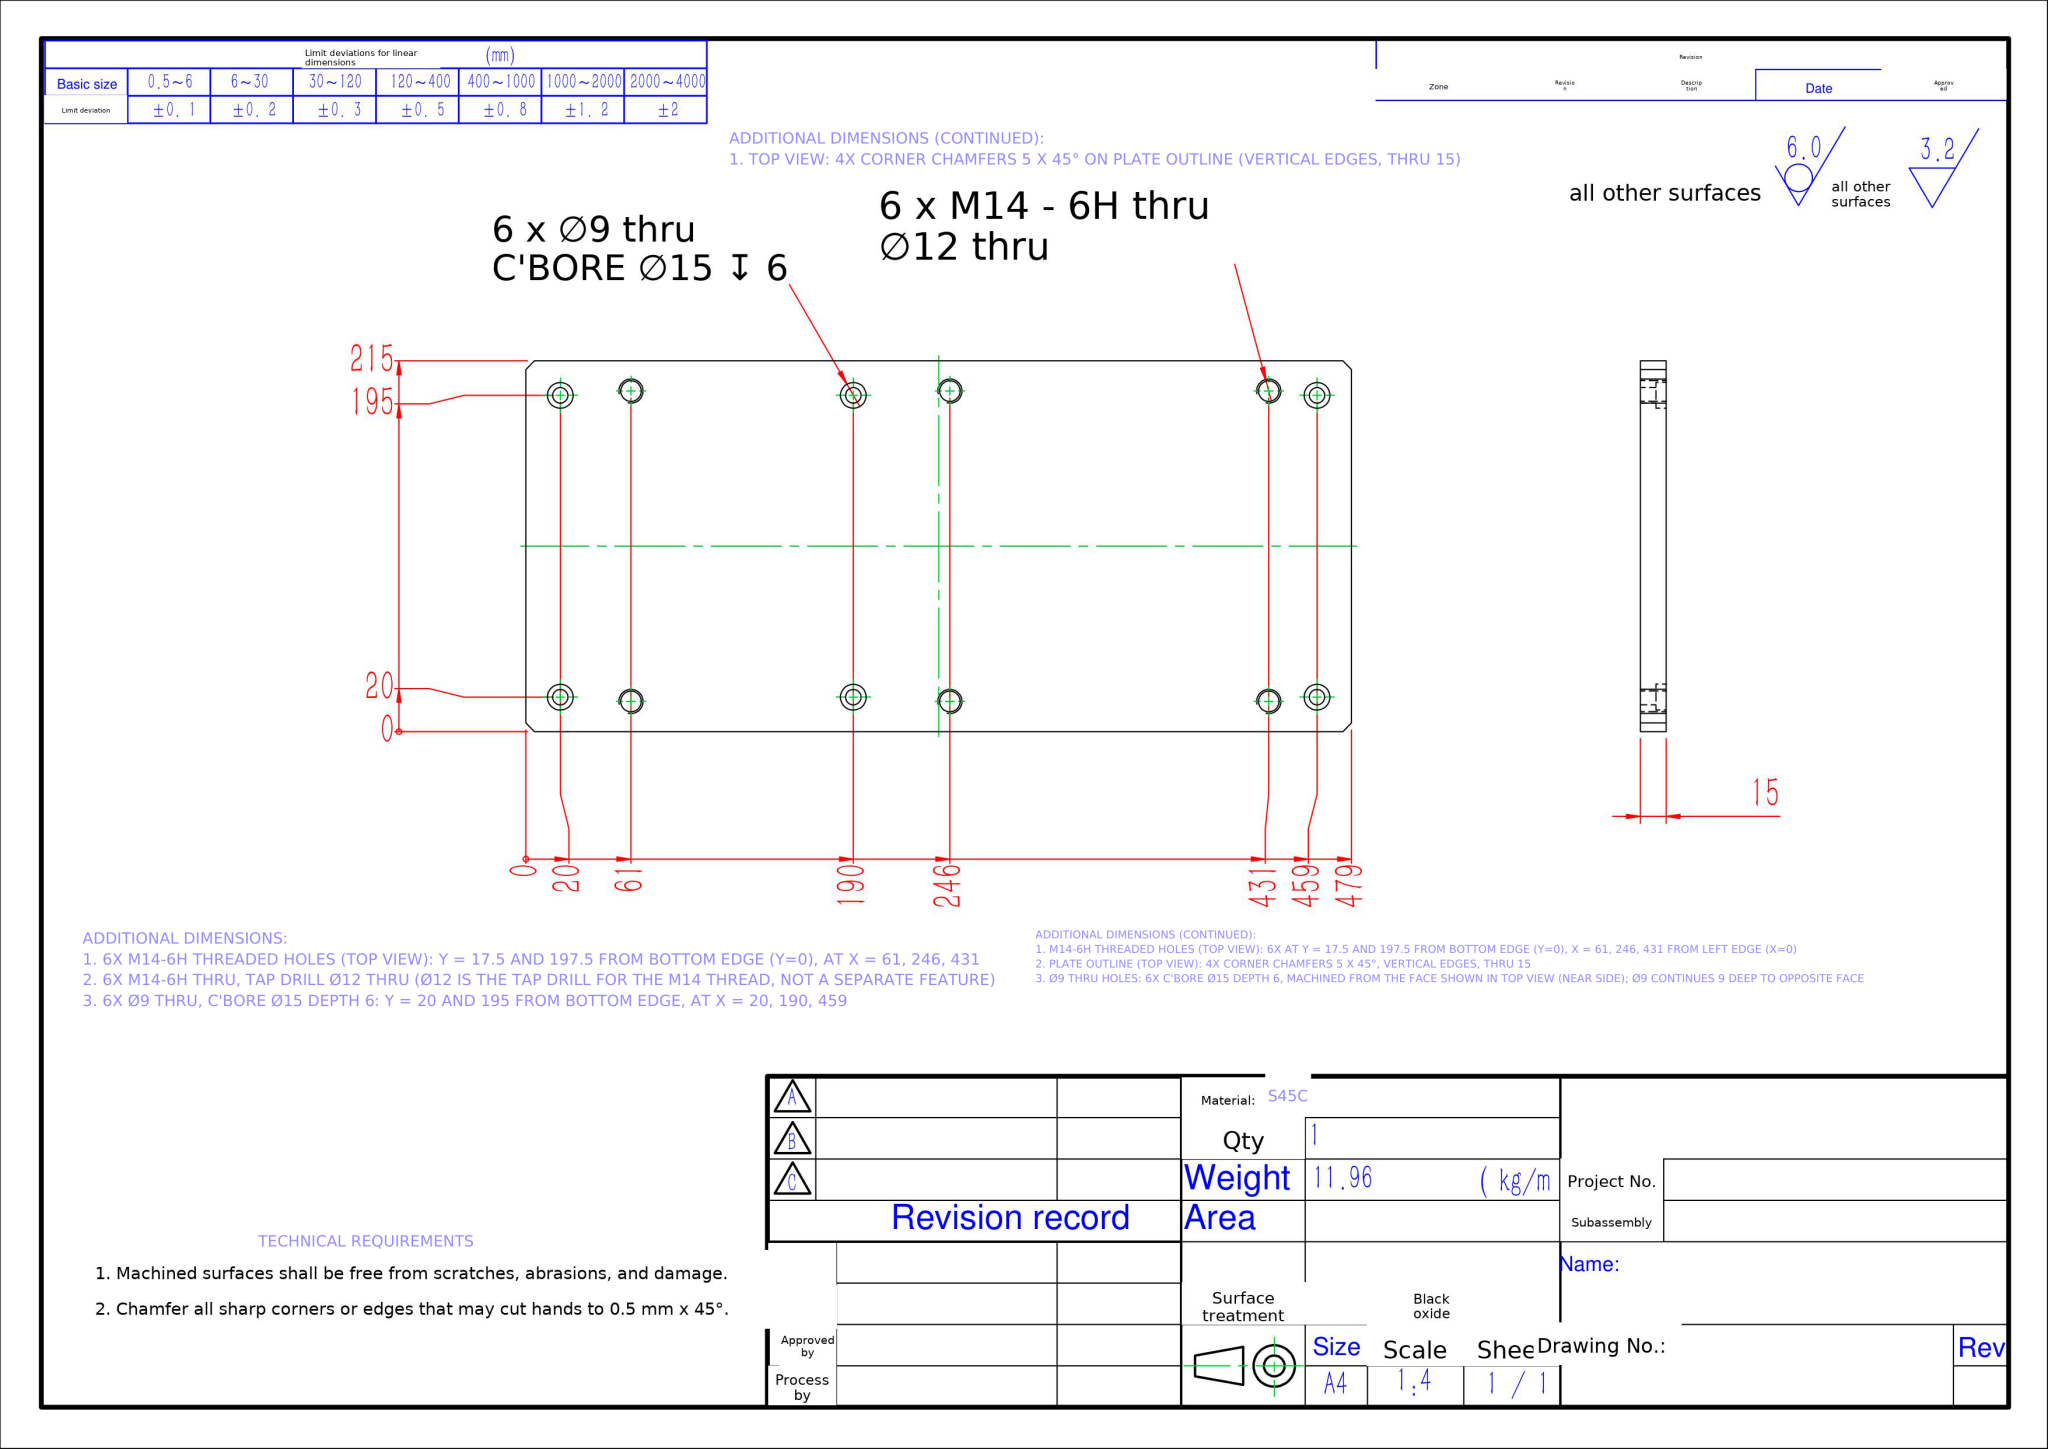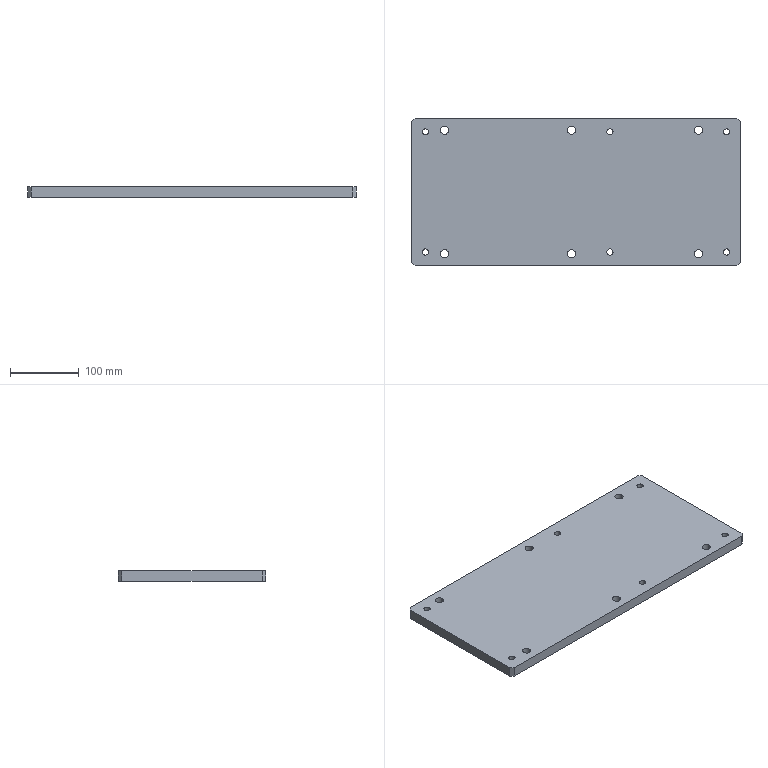Part | NX | mm | 1 solid | 52 faces | box 479 x 215 x 15 mm | volume 1524049 mm3 | cylinder 36 | plane 16 | commonest cylinder face diameters 15 x12 9 x12 12 x12